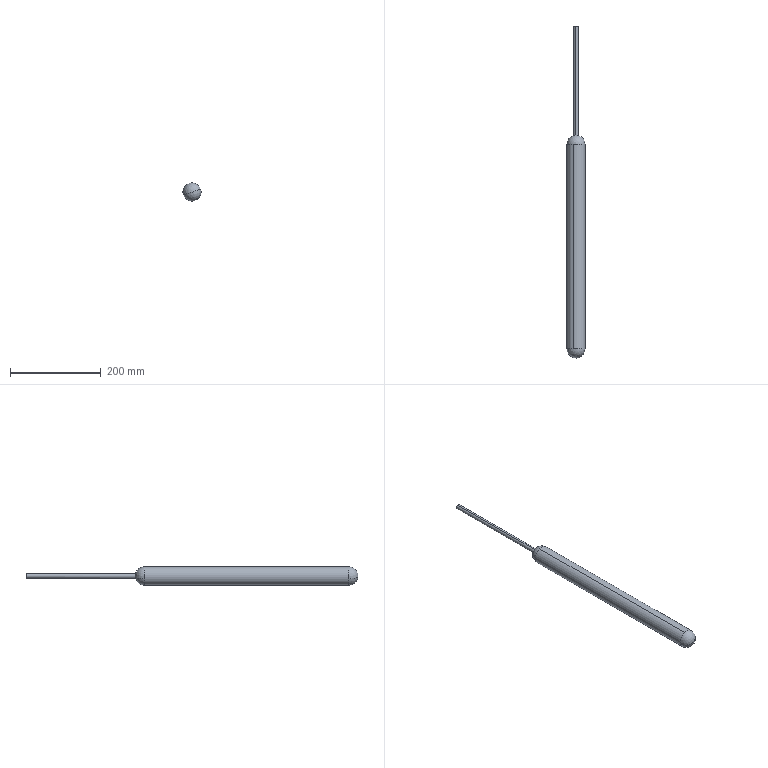Component | SolidWorks | InsectTrapLamp-1_LampTube-1 | 1 solid | 9 faces | box 40 x 730 x 40 mm | volume 617871 mm3 | cylinder 4 | sphere 4 | plane 1 | commonest cylinder face diameters 10 x2 40 x2
build123d program:
from build123d import *

# Parameters (mm, degrees)
SKETCH2_R           = 5
BOSS_EXTRUDE1_DEPTH = 260


with BuildPart() as part:
    # Sketch1 → Revolve1 (revolve)
    with BuildSketch(Plane.XY, mode=Mode.PRIVATE) as revolve1_sk:
        with BuildLine():
            Line((0, -20), (450, -20))
            ThreePointArc((450, -20), (464.142, -14.142), (470, 0))
            Line((470, 0), (-20, 0))
            ThreePointArc((-20, 0), (-14.142, -14.142), (0, -20))
        make_face()
    revolve(revolve1_sk.sketch.rotate(Axis((0, 0, 0), (1, 0, 0)), 270), axis=Axis((0, 0, 0), (1, 0, 0)))

    # Sketch2 → Boss-Extrude1 (add)
    with BuildSketch(Plane(origin=(0, 0, 0), x_dir=(0, 0, -1), z_dir=(1, 0, 0))):
        Circle(SKETCH2_R)
    extrude(amount=-BOSS_EXTRUDE1_DEPTH)


solid = part.part

# Placed as in the assembly
solid = solid.moved(Location((0, 1370, 0), (0, 0, -90)))
STEP:
#1=COLOUR_RGB('',0.7922,0.8196,0.9333);
#2=FILL_AREA_STYLE_COLOUR('',#1);
#3=FILL_AREA_STYLE('',(#2));
#4=SURFACE_STYLE_FILL_AREA(#3);
#5=SURFACE_SIDE_STYLE('',(#4));
#6=SURFACE_STYLE_USAGE(.BOTH.,#5);
#7=PRESENTATION_STYLE_ASSIGNMENT((#6));
#8=CARTESIAN_POINT('',(0.05823,64.173,-0.188));
#9=VERTEX_POINT('',#8);
#10=CARTESIAN_POINT('',(-0.05823,64.173,0.188));
#11=VERTEX_POINT('',#10);
#12=CARTESIAN_POINT('',(0.,64.173,-0.));
#13=DIRECTION('',(0.,-1.,0.));
#14=DIRECTION('',(0.2958,0.,-0.9552));
#15=AXIS2_PLACEMENT_3D('',#12,#13,#14);
#16=CIRCLE('',#15,0.1969);
#17=EDGE_CURVE('',#9,#11,#16,.T.);
#18=ORIENTED_EDGE('',*,*,#17,.T.);
#19=CARTESIAN_POINT('',(-0.05823,54.699,0.188));
#20=VERTEX_POINT('',#19);
#21=CARTESIAN_POINT('',(-0.05823,64.173,0.188));
#22=DIRECTION('',(0.,-1.,0.));
#23=VECTOR('',#22,39.37);
#24=LINE('',#21,#23);
#25=EDGE_CURVE('',#11,#20,#24,.T.);
#26=ORIENTED_EDGE('',*,*,#25,.T.);
#27=CARTESIAN_POINT('',(0.188,54.699,0.05823));
#28=VERTEX_POINT('',#27);
#29=CARTESIAN_POINT('',(0.,54.699,-0.));
#30=DIRECTION('',(0.,1.,0.));
#31=DIRECTION('',(0.2958,0.,-0.9552));
#32=AXIS2_PLACEMENT_3D('',#29,#30,#31);
#33=CIRCLE('',#32,0.1969);
#34=EDGE_CURVE('',#20,#28,#33,.T.);
#35=ORIENTED_EDGE('',*,*,#34,.T.);
#36=CARTESIAN_POINT('',(0.05823,54.699,-0.188));
#37=VERTEX_POINT('',#36);
#38=CARTESIAN_POINT('',(0.,54.699,-0.));
#39=DIRECTION('',(0.,1.,0.));
#40=DIRECTION('',(0.2958,0.,-0.9552));
#41=AXIS2_PLACEMENT_3D('',#38,#39,#40);
#42=CIRCLE('',#41,0.1969);
#43=EDGE_CURVE('',#28,#37,#42,.T.);
#44=ORIENTED_EDGE('',*,*,#43,.T.);
#45=CARTESIAN_POINT('',(0.05823,64.173,-0.188));
#46=DIRECTION('',(0.,-1.,0.));
#47=VECTOR('',#46,39.37);
#48=LINE('',#45,#47);
#49=EDGE_CURVE('',#9,#37,#48,.T.);
#50=ORIENTED_EDGE('',*,*,#49,.F.);
#51=EDGE_LOOP('',(#18,#26,#35,#44,#50));
#52=FACE_OUTER_BOUND('',#51,.T.);
#53=CARTESIAN_POINT('',(0.,64.173,-0.));
#54=DIRECTION('',(0.,-1.,0.));
#55=DIRECTION('',(0.2958,0.,-0.9552));
#56=AXIS2_PLACEMENT_3D('',#53,#54,#55);
#57=CYLINDRICAL_SURFACE('',#56,0.1969);
#58=ADVANCED_FACE('',(#52),#57,.T.);
#59=CARTESIAN_POINT('',(0.,35.433,-0.));
#60=VERTEX_POINT('',#59);
#61=CARTESIAN_POINT('',(-0.7522,36.22,-0.2329));
#62=VERTEX_POINT('',#61);
#63=CARTESIAN_POINT('',(0.,36.22,-0.));
#64=DIRECTION('',(0.2958,0.,-0.9552));
#65=DIRECTION('',(-0.9552,0.,-0.2958));
#66=AXIS2_PLACEMENT_3D('',#63,#64,#65);
#67=CIRCLE('',#66,0.7874);
#68=EDGE_CURVE('',#60,#62,#67,.T.);
#69=ORIENTED_EDGE('',*,*,#68,.F.);
#70=CARTESIAN_POINT('',(0.7522,36.22,0.2329));
#71=VERTEX_POINT('',#70);
#72=CARTESIAN_POINT('',(0.,36.22,-0.));
#73=DIRECTION('',(-0.2958,0.,0.9552));
#74=DIRECTION('',(0.9552,0.,0.2958));
#75=AXIS2_PLACEMENT_3D('',#72,#73,#74);
#76=CIRCLE('',#75,0.7874);
#77=EDGE_CURVE('',#60,#71,#76,.T.);
#78=ORIENTED_EDGE('',*,*,#77,.T.);
#79=CARTESIAN_POINT('',(-0.2329,36.22,0.7522));
#80=VERTEX_POINT('',#79);
#81=CARTESIAN_POINT('',(0.,36.22,-0.));
#82=DIRECTION('',(0.,1.,0.));
#83=DIRECTION('',(-0.2958,0.,0.9552));
#84=AXIS2_PLACEMENT_3D('',#81,#82,#83);
#85=CIRCLE('',#84,0.7874);
#86=EDGE_CURVE('',#80,#71,#85,.T.);
#87=ORIENTED_EDGE('',*,*,#86,.F.);
#88=CARTESIAN_POINT('',(0.,36.22,-0.));
#89=DIRECTION('',(0.,1.,0.));
#90=DIRECTION('',(-0.2958,0.,0.9552));
#91=AXIS2_PLACEMENT_3D('',#88,#89,#90);
#92=CIRCLE('',#91,0.7874);
#93=EDGE_CURVE('',#62,#80,#92,.T.);
#94=ORIENTED_EDGE('',*,*,#93,.F.);
#95=EDGE_LOOP('',(#69,#78,#87,#94));
#96=FACE_OUTER_BOUND('',#95,.T.);
#97=CARTESIAN_POINT('',(0.,36.22,-0.));
#98=DIRECTION('',(-0.2958,0.,0.9552));
#99=DIRECTION('',(-0.9552,0.,-0.2958));
#100=AXIS2_PLACEMENT_3D('',#97,#98,#99);
#101=SPHERICAL_SURFACE('',#100,0.7874);
#102=ADVANCED_FACE('',(#96),#101,.T.);
#103=ORIENTED_EDGE('',*,*,#86,.T.);
#104=CARTESIAN_POINT('',(0.2329,36.22,-0.7522));
#105=VERTEX_POINT('',#104);
#106=CARTESIAN_POINT('',(0.,36.22,-0.));
#107=DIRECTION('',(0.,1.,0.));
#108=DIRECTION('',(-0.2958,0.,0.9552));
#109=AXIS2_PLACEMENT_3D('',#106,#107,#108);
#110=CIRCLE('',#109,0.7874);
#111=EDGE_CURVE('',#71,#105,#110,.T.);
#112=ORIENTED_EDGE('',*,*,#111,.T.);
#113=CARTESIAN_POINT('',(0.2329,53.937,-0.7522));
#114=VERTEX_POINT('',#113);
#115=CARTESIAN_POINT('',(0.2329,53.937,-0.7522));
#116=DIRECTION('',(0.,1.,0.));
#117=VECTOR('',#116,39.37);
#118=LINE('',#115,#117);
#119=EDGE_CURVE('',#105,#114,#118,.T.);
#120=ORIENTED_EDGE('',*,*,#119,.T.);
#121=CARTESIAN_POINT('',(0.7522,53.937,0.2329));
#122=VERTEX_POINT('',#121);
#123=CARTESIAN_POINT('',(0.,53.937,-0.));
#124=DIRECTION('',(0.,1.,0.));
#125=DIRECTION('',(-0.2958,0.,0.9552));
#126=AXIS2_PLACEMENT_3D('',#123,#124,#125);
#127=CIRCLE('',#126,0.7874);
#128=EDGE_CURVE('',#122,#114,#127,.T.);
#129=ORIENTED_EDGE('',*,*,#128,.F.);
#130=CARTESIAN_POINT('',(-0.2329,53.937,0.7522));
#131=VERTEX_POINT('',#130);
#132=CARTESIAN_POINT('',(0.,53.937,-0.));
#133=DIRECTION('',(0.,1.,0.));
#134=DIRECTION('',(-0.2958,0.,0.9552));
#135=AXIS2_PLACEMENT_3D('',#132,#133,#134);
#136=CIRCLE('',#135,0.7874);
#137=EDGE_CURVE('',#131,#122,#136,.T.);
#138=ORIENTED_EDGE('',*,*,#137,.F.);
#139=CARTESIAN_POINT('',(-0.2329,53.937,0.7522));
#140=DIRECTION('',(0.,1.,0.));
#141=VECTOR('',#140,39.37);
#142=LINE('',#139,#141);
#143=EDGE_CURVE('',#80,#131,#142,.T.);
#144=ORIENTED_EDGE('',*,*,#143,.F.);
#145=EDGE_LOOP('',(#103,#112,#120,#129,#138,#144));
#146=FACE_OUTER_BOUND('',#145,.T.);
#147=CARTESIAN_POINT('',(0.,53.937,-0.));
#148=DIRECTION('',(0.,1.,0.));
#149=DIRECTION('',(-0.2958,0.,0.9552));
#150=AXIS2_PLACEMENT_3D('',#147,#148,#149);
#151=CYLINDRICAL_SURFACE('',#150,0.7874);
#152=ADVANCED_FACE('',(#146),#151,.T.);
#153=ORIENTED_EDGE('',*,*,#128,.T.);
#154=CARTESIAN_POINT('',(-0.7522,53.937,-0.2329));
#155=VERTEX_POINT('',#154);
#156=CARTESIAN_POINT('',(0.,53.937,-0.));
#157=DIRECTION('',(0.,1.,0.));
#158=DIRECTION('',(-0.2958,0.,0.9552));
#159=AXIS2_PLACEMENT_3D('',#156,#157,#158);
#160=CIRCLE('',#159,0.7874);
#161=EDGE_CURVE('',#114,#155,#160,.T.);
#162=ORIENTED_EDGE('',*,*,#161,.T.);
#163=CARTESIAN_POINT('',(-0.188,54.699,-0.05823));
#164=VERTEX_POINT('',#163);
#165=CARTESIAN_POINT('',(0.,53.937,-0.));
#166=DIRECTION('',(0.2958,0.,-0.9552));
#167=DIRECTION('',(-0.9552,0.,-0.2958));
#168=AXIS2_PLACEMENT_3D('',#165,#166,#167);
#169=CIRCLE('',#168,0.7874);
#170=EDGE_CURVE('',#155,#164,#169,.T.);
#171=ORIENTED_EDGE('',*,*,#170,.T.);
#172=CARTESIAN_POINT('',(0.,54.699,-0.));
#173=DIRECTION('',(0.,1.,0.));
#174=DIRECTION('',(0.2958,0.,-0.9552));
#175=AXIS2_PLACEMENT_3D('',#172,#173,#174);
#176=CIRCLE('',#175,0.1969);
#177=EDGE_CURVE('',#37,#164,#176,.T.);
#178=ORIENTED_EDGE('',*,*,#177,.F.);
#179=ORIENTED_EDGE('',*,*,#43,.F.);
#180=CARTESIAN_POINT('',(0.,53.937,-0.));
#181=DIRECTION('',(-0.2958,0.,0.9552));
#182=DIRECTION('',(0.9552,0.,0.2958));
#183=AXIS2_PLACEMENT_3D('',#180,#181,#182);
#184=CIRCLE('',#183,0.7874);
#185=EDGE_CURVE('',#122,#28,#184,.T.);
#186=ORIENTED_EDGE('',*,*,#185,.F.);
#187=EDGE_LOOP('',(#153,#162,#171,#178,#179,#186));
#188=FACE_OUTER_BOUND('',#187,.T.);
#189=CARTESIAN_POINT('',(0.,53.937,-0.));
#190=DIRECTION('',(0.2958,0.,-0.9552));
#191=DIRECTION('',(0.9552,0.,0.2958));
#192=AXIS2_PLACEMENT_3D('',#189,#190,#191);
#193=SPHERICAL_SURFACE('',#192,0.7874);
#194=ADVANCED_FACE('',(#188),#193,.T.);
#195=ORIENTED_EDGE('',*,*,#170,.F.);
#196=CARTESIAN_POINT('',(0.,53.937,-0.));
#197=DIRECTION('',(0.,1.,0.));
#198=DIRECTION('',(-0.2958,0.,0.9552));
#199=AXIS2_PLACEMENT_3D('',#196,#197,#198);
#200=CIRCLE('',#199,0.7874);
#201=EDGE_CURVE('',#155,#131,#200,.T.);
#202=ORIENTED_EDGE('',*,*,#201,.T.);
#203=ORIENTED_EDGE('',*,*,#137,.T.);
#204=ORIENTED_EDGE('',*,*,#185,.T.);
#205=ORIENTED_EDGE('',*,*,#34,.F.);
#206=CARTESIAN_POINT('',(0.,54.699,-0.));
#207=DIRECTION('',(0.,1.,0.));
#208=DIRECTION('',(0.2958,0.,-0.9552));
#209=AXIS2_PLACEMENT_3D('',#206,#207,#208);
#210=CIRCLE('',#209,0.1969);
#211=EDGE_CURVE('',#164,#20,#210,.T.);
#212=ORIENTED_EDGE('',*,*,#211,.F.);
#213=EDGE_LOOP('',(#195,#202,#203,#204,#205,#212));
#214=FACE_OUTER_BOUND('',#213,.T.);
#215=CARTESIAN_POINT('',(0.,53.937,-0.));
#216=DIRECTION('',(0.2958,0.,-0.9552));
#217=DIRECTION('',(0.9552,0.,0.2958));
#218=AXIS2_PLACEMENT_3D('',#215,#216,#217);
#219=SPHERICAL_SURFACE('',#218,0.7874);
#220=ADVANCED_FACE('',(#214),#219,.T.);
#221=ORIENTED_EDGE('',*,*,#119,.F.);
#222=CARTESIAN_POINT('',(0.,36.22,-0.));
#223=DIRECTION('',(0.,1.,0.));
#224=DIRECTION('',(-0.2958,0.,0.9552));
#225=AXIS2_PLACEMENT_3D('',#222,#223,#224);
#226=CIRCLE('',#225,0.7874);
#227=EDGE_CURVE('',#105,#62,#226,.T.);
#228=ORIENTED_EDGE('',*,*,#227,.T.);
#229=ORIENTED_EDGE('',*,*,#93,.T.);
#230=ORIENTED_EDGE('',*,*,#143,.T.);
#231=ORIENTED_EDGE('',*,*,#201,.F.);
#232=ORIENTED_EDGE('',*,*,#161,.F.);
#233=EDGE_LOOP('',(#221,#228,#229,#230,#231,#232));
#234=FACE_OUTER_BOUND('',#233,.T.);
#235=CARTESIAN_POINT('',(0.,53.937,-0.));
#236=DIRECTION('',(0.,1.,0.));
#237=DIRECTION('',(-0.2958,0.,0.9552));
#238=AXIS2_PLACEMENT_3D('',#235,#236,#237);
#239=CYLINDRICAL_SURFACE('',#238,0.7874);
#240=ADVANCED_FACE('',(#234),#239,.T.);
#241=ORIENTED_EDGE('',*,*,#77,.F.);
#242=ORIENTED_EDGE('',*,*,#68,.T.);
#243=ORIENTED_EDGE('',*,*,#227,.F.);
#244=ORIENTED_EDGE('',*,*,#111,.F.);
#245=EDGE_LOOP('',(#241,#242,#243,#244));
#246=FACE_OUTER_BOUND('',#245,.T.);
#247=CARTESIAN_POINT('',(0.,36.22,-0.));
#248=DIRECTION('',(-0.2958,0.,0.9552));
#249=DIRECTION('',(-0.9552,0.,-0.2958));
#250=AXIS2_PLACEMENT_3D('',#247,#248,#249);
#251=SPHERICAL_SURFACE('',#250,0.7874);
#252=ADVANCED_FACE('',(#246),#251,.T.);
#253=ORIENTED_EDGE('',*,*,#25,.F.);
#254=CARTESIAN_POINT('',(0.,64.173,-0.));
#255=DIRECTION('',(0.,-1.,0.));
#256=DIRECTION('',(0.2958,0.,-0.9552));
#257=AXIS2_PLACEMENT_3D('',#254,#255,#256);
#258=CIRCLE('',#257,0.1969);
#259=EDGE_CURVE('',#11,#9,#258,.T.);
#260=ORIENTED_EDGE('',*,*,#259,.T.);
#261=ORIENTED_EDGE('',*,*,#49,.T.);
#262=ORIENTED_EDGE('',*,*,#177,.T.);
#263=ORIENTED_EDGE('',*,*,#211,.T.);
#264=EDGE_LOOP('',(#253,#260,#261,#262,#263));
#265=FACE_OUTER_BOUND('',#264,.T.);
#266=CARTESIAN_POINT('',(0.,64.173,-0.));
#267=DIRECTION('',(0.,-1.,0.));
#268=DIRECTION('',(0.2958,0.,-0.9552));
#269=AXIS2_PLACEMENT_3D('',#266,#267,#268);
#270=CYLINDRICAL_SURFACE('',#269,0.1969);
#271=ADVANCED_FACE('',(#265),#270,.T.);
#272=ORIENTED_EDGE('',*,*,#17,.F.);
#273=ORIENTED_EDGE('',*,*,#259,.F.);
#274=EDGE_LOOP('',(#272,#273));
#275=FACE_OUTER_BOUND('',#274,.T.);
#276=CARTESIAN_POINT('',(0.,64.173,-0.));
#277=DIRECTION('',(0.,-1.,0.));
#278=DIRECTION('',(0.2958,0.,-0.9552));
#279=AXIS2_PLACEMENT_3D('',#276,#277,#278);
#280=PLANE('',#279);
#281=ADVANCED_FACE('',(#275),#280,.F.);
#282=CLOSED_SHELL('',(#58,#102,#152,#194,#220,#240,#252,#271,#281));
#283=MANIFOLD_SOLID_BREP('',#282);
#284=STYLED_ITEM('',(#7),#283);
#285=(LENGTH_UNIT()NAMED_UNIT(*)SI_UNIT($,.METRE.));
#286=LENGTH_MEASURE_WITH_UNIT(LENGTH_MEASURE(0.0254),#285);
#287=DIMENSIONAL_EXPONENTS(1.,0.,0.,0.,0.,0.,0.);
#288=(CONVERSION_BASED_UNIT('',#286)LENGTH_UNIT()NAMED_UNIT(#287));
#289=UNCERTAINTY_MEASURE_WITH_UNIT(LENGTH_MEASURE(0.00001),#288,'','');
#290=(NAMED_UNIT(*)PLANE_ANGLE_UNIT()SI_UNIT($,.RADIAN.));
#291=(NAMED_UNIT(*)SI_UNIT($,.STERADIAN.)SOLID_ANGLE_UNIT());
#292=(GEOMETRIC_REPRESENTATION_CONTEXT(3)GLOBAL_UNCERTAINTY_ASSIGNED_CONTEXT((#289))GLOBAL_UNIT_ASSIGNED_CONTEXT((#288,#290,#291))REPRESENTATION_CONTEXT('',''));
#293=MECHANICAL_DESIGN_GEOMETRIC_PRESENTATION_REPRESENTATION('',(#284),#292);
#294=PRESENTATION_LAYER_ASSIGNMENT('','',(#284));
#295=CARTESIAN_POINT('',(0.,0.,0.));
#296=DIRECTION('',(0.,0.,1.));
#297=DIRECTION('',(1.,0.,0.));
#298=AXIS2_PLACEMENT_3D('',#295,#296,#297);
#299=(LENGTH_UNIT()NAMED_UNIT(*)SI_UNIT($,.METRE.));
#300=LENGTH_MEASURE_WITH_UNIT(LENGTH_MEASURE(0.0254),#299);
#301=DIMENSIONAL_EXPONENTS(1.,0.,0.,0.,0.,0.,0.);
#302=(CONVERSION_BASED_UNIT('',#300)LENGTH_UNIT()NAMED_UNIT(#301));
#303=UNCERTAINTY_MEASURE_WITH_UNIT(LENGTH_MEASURE(0.00001),#302,'','');
#304=(NAMED_UNIT(*)PLANE_ANGLE_UNIT()SI_UNIT($,.RADIAN.));
#305=(NAMED_UNIT(*)SI_UNIT($,.STERADIAN.)SOLID_ANGLE_UNIT());
#306=(GEOMETRIC_REPRESENTATION_CONTEXT(3)GLOBAL_UNCERTAINTY_ASSIGNED_CONTEXT((#303))GLOBAL_UNIT_ASSIGNED_CONTEXT((#302,#304,#305))REPRESENTATION_CONTEXT('',''));
#307=ADVANCED_BREP_SHAPE_REPRESENTATION('',(#283,#298),#306);